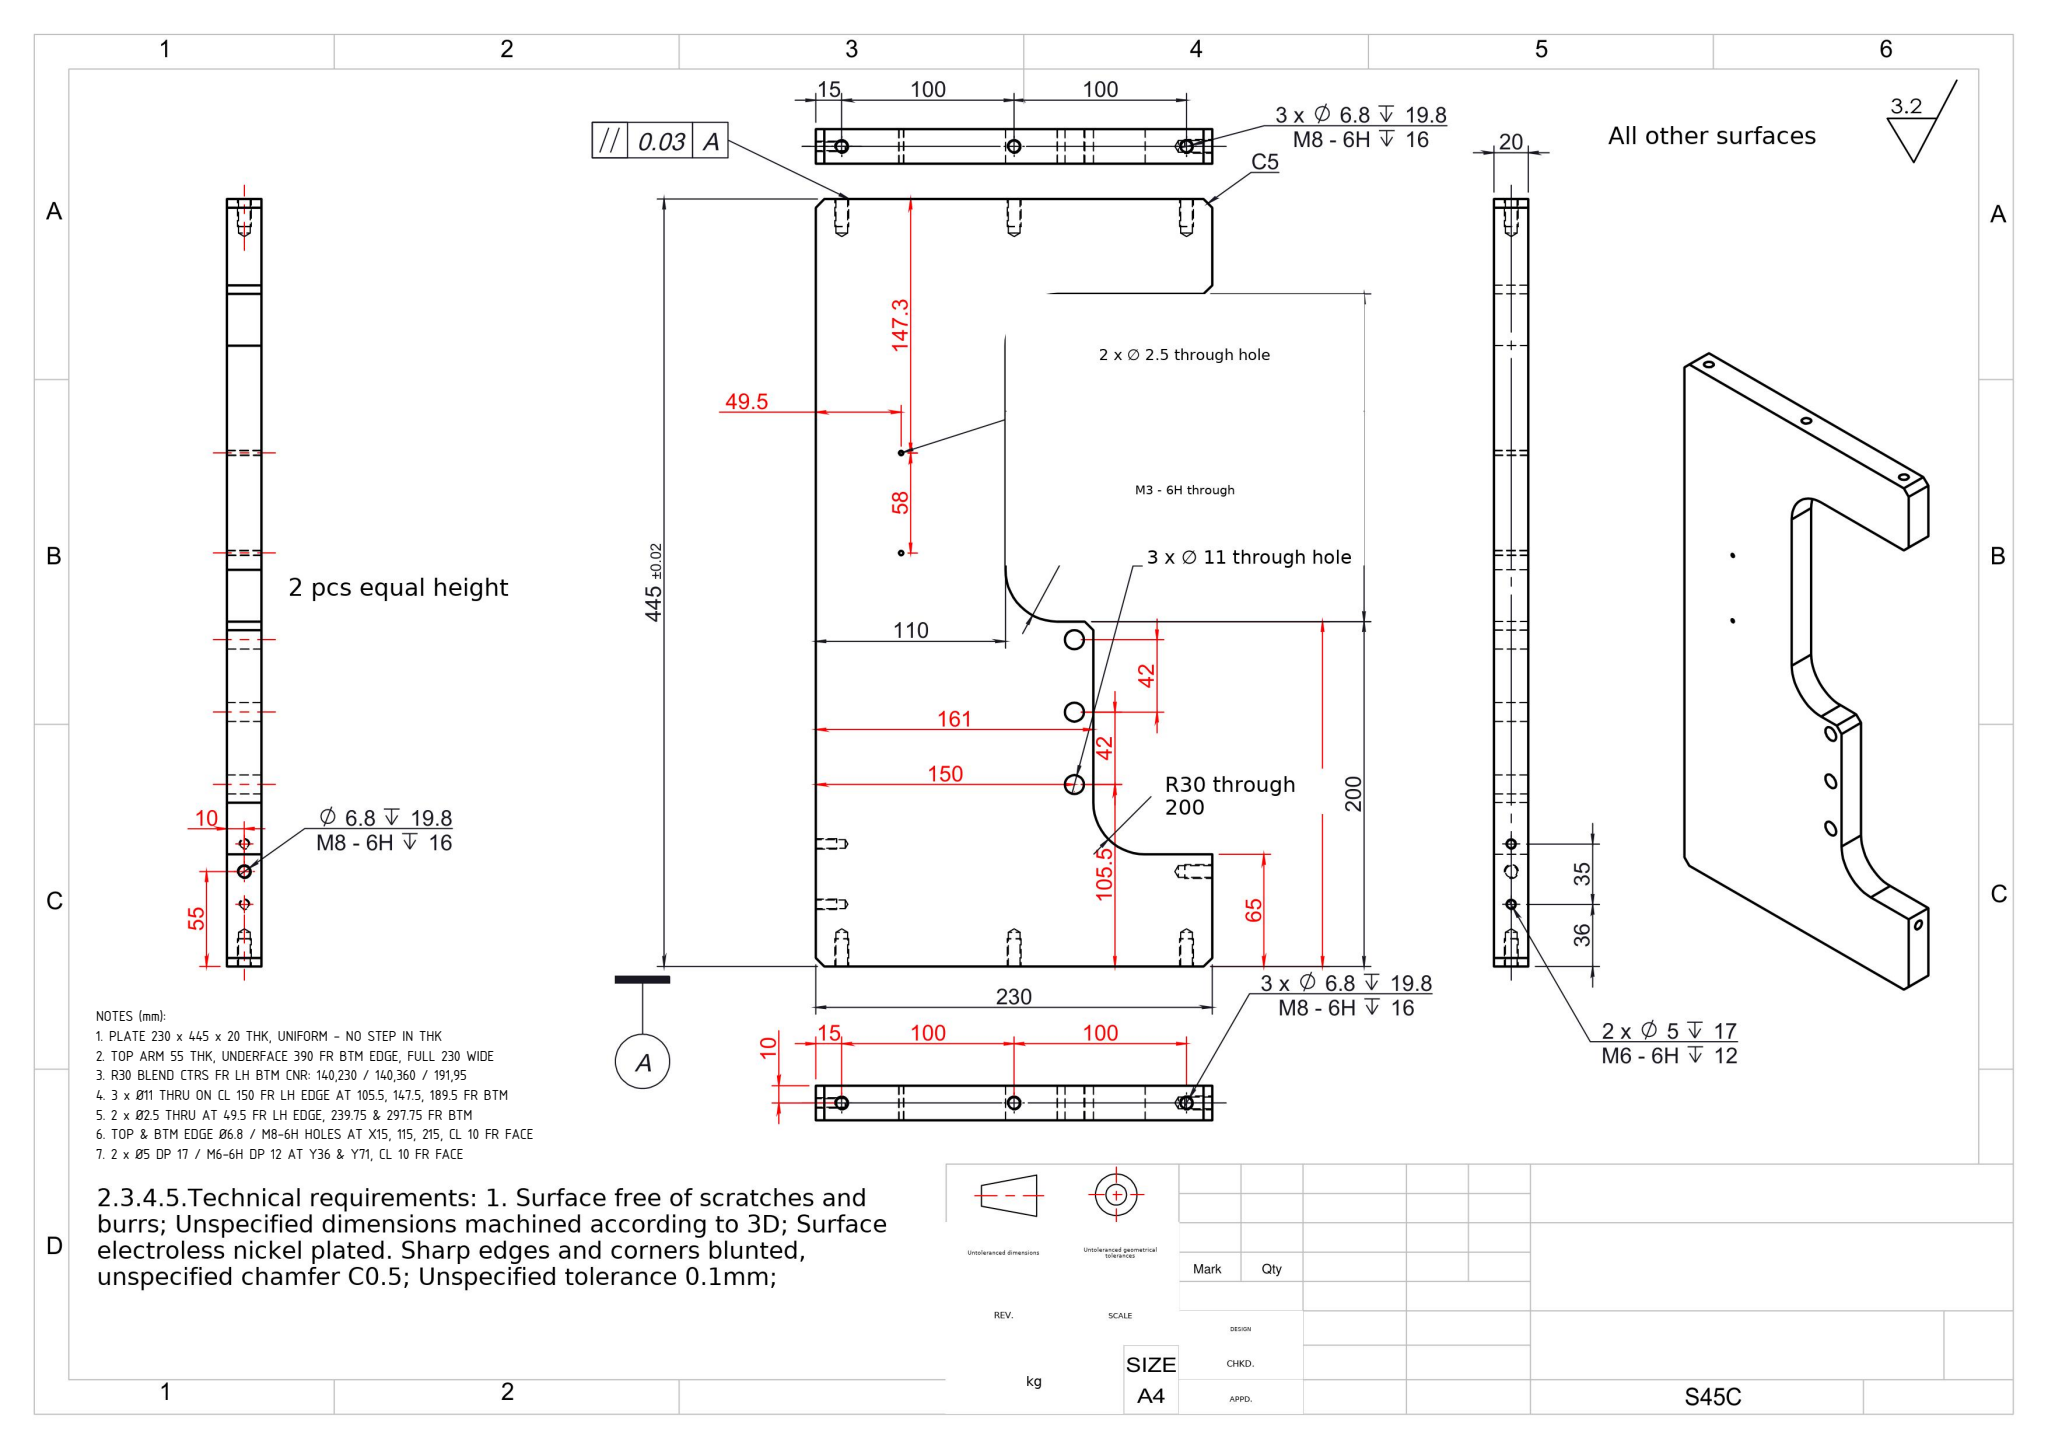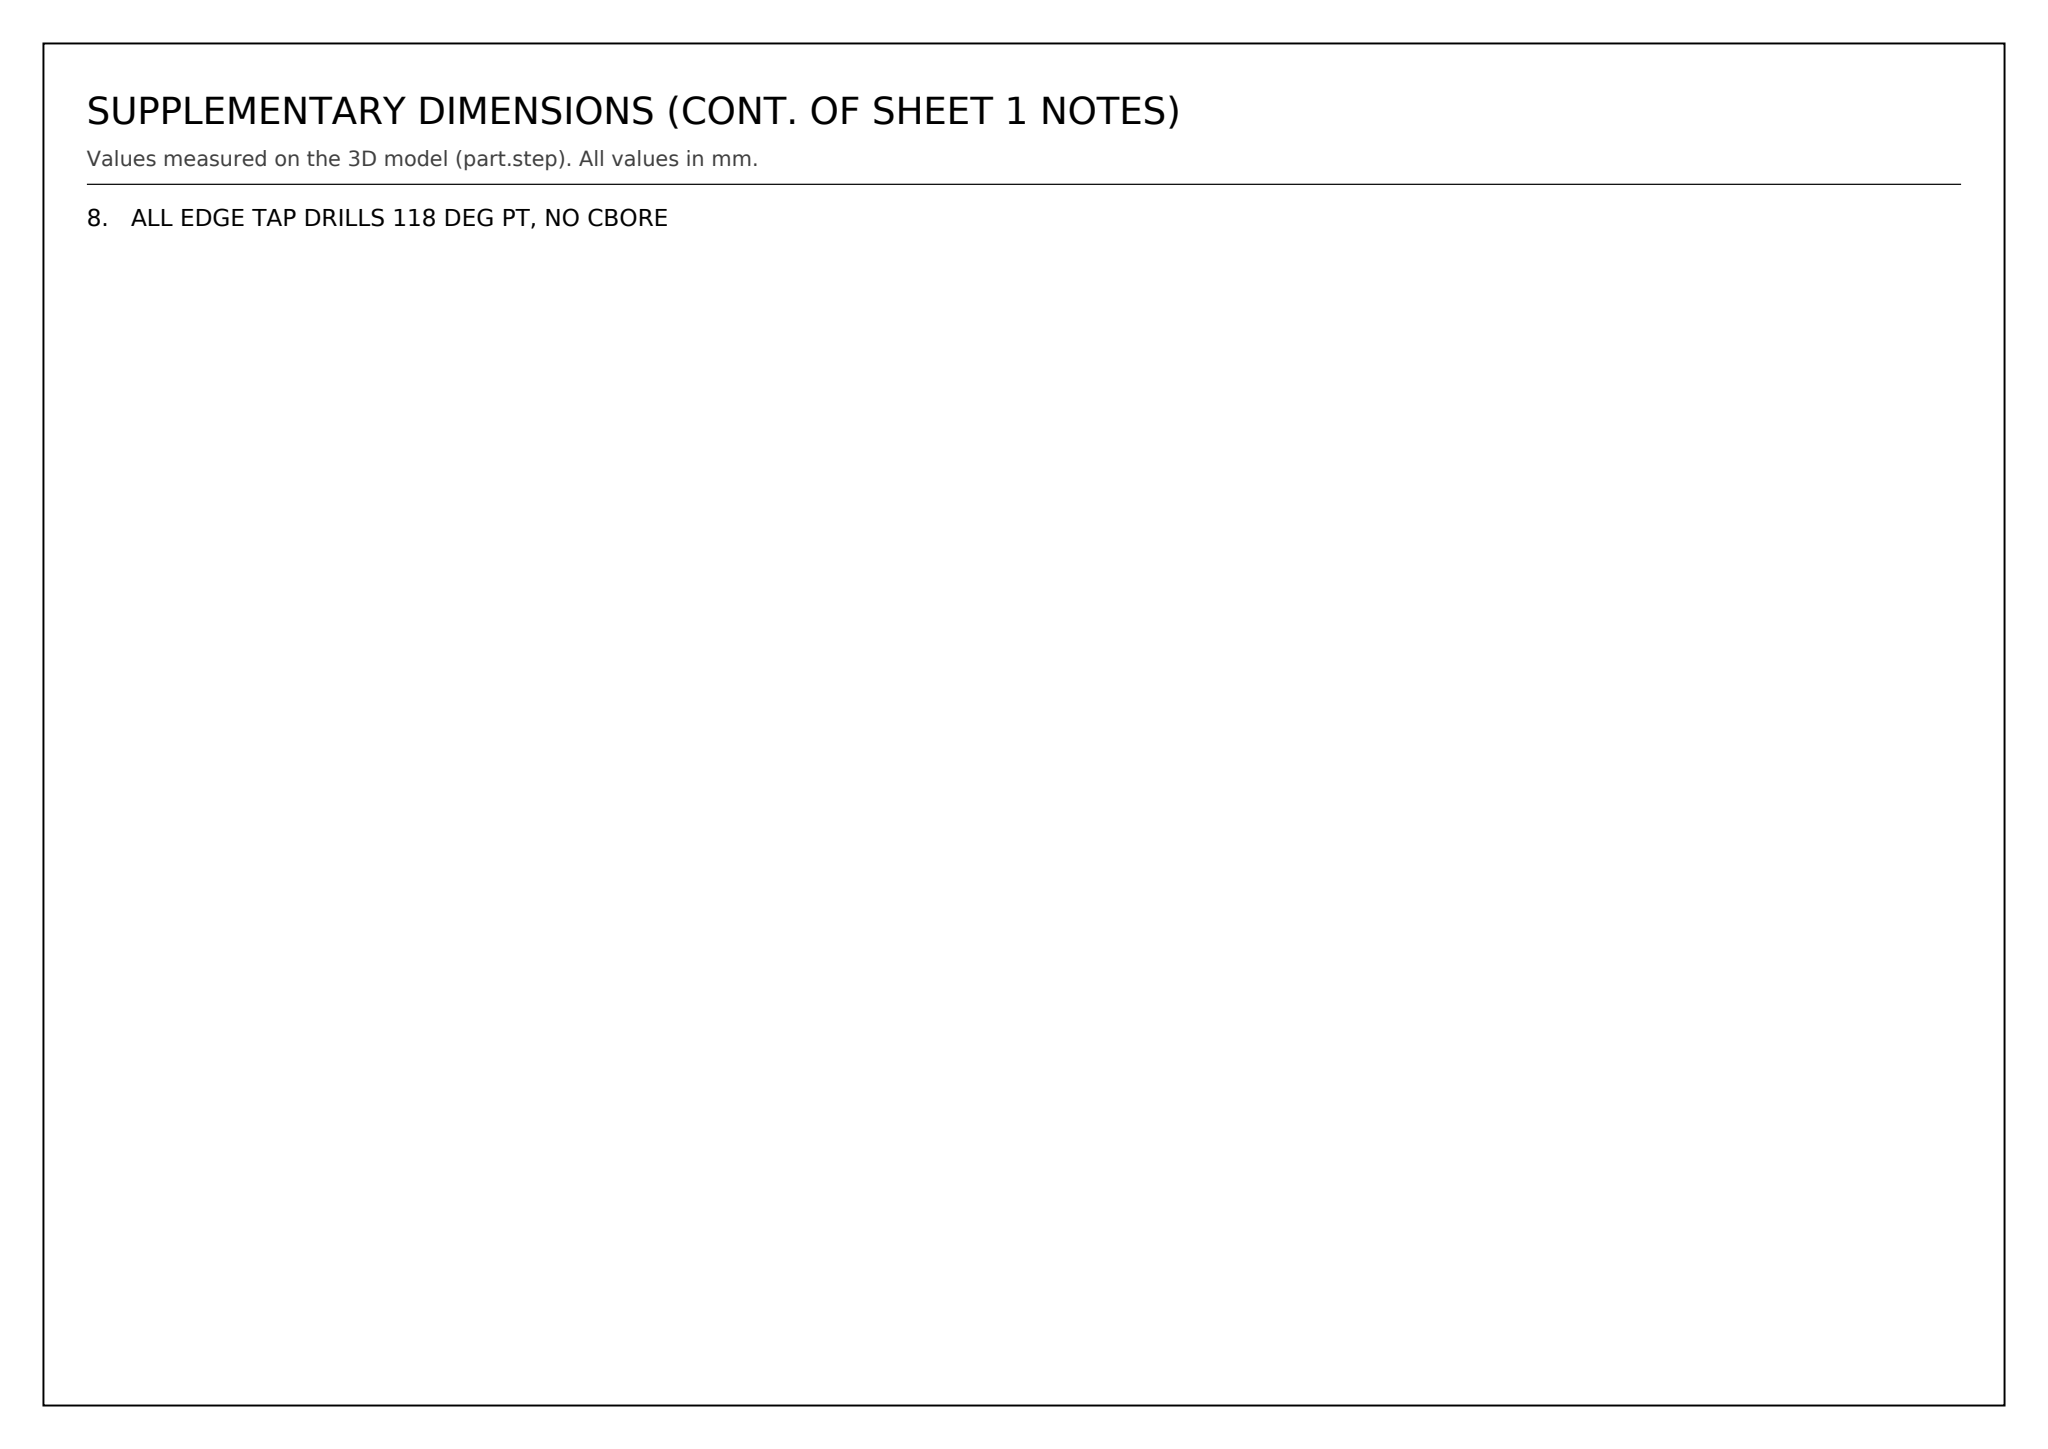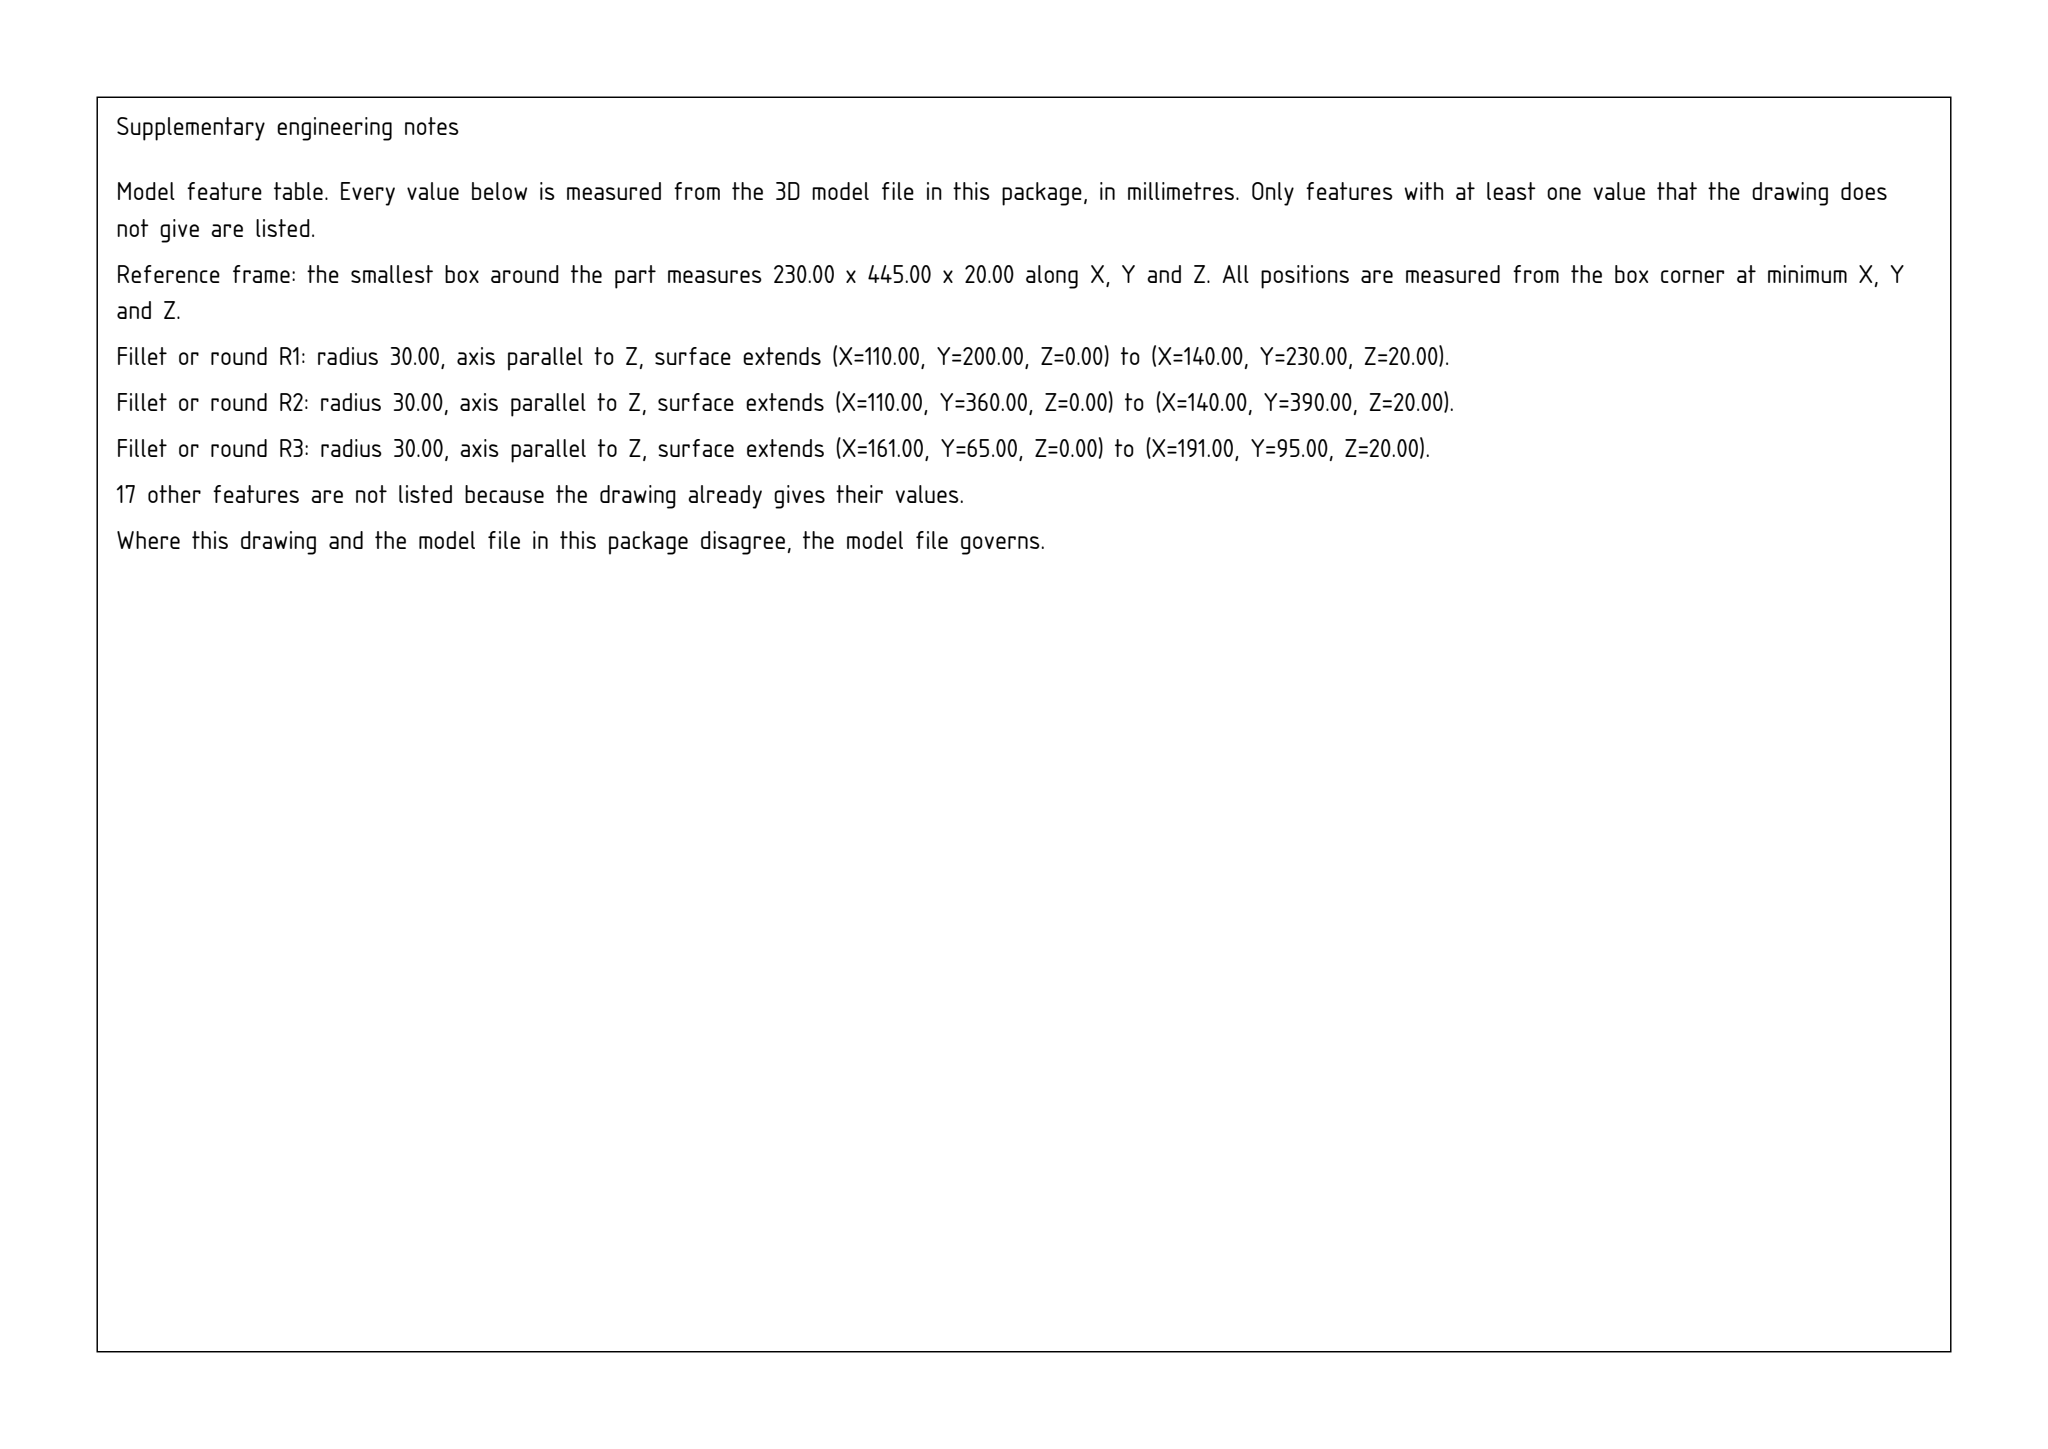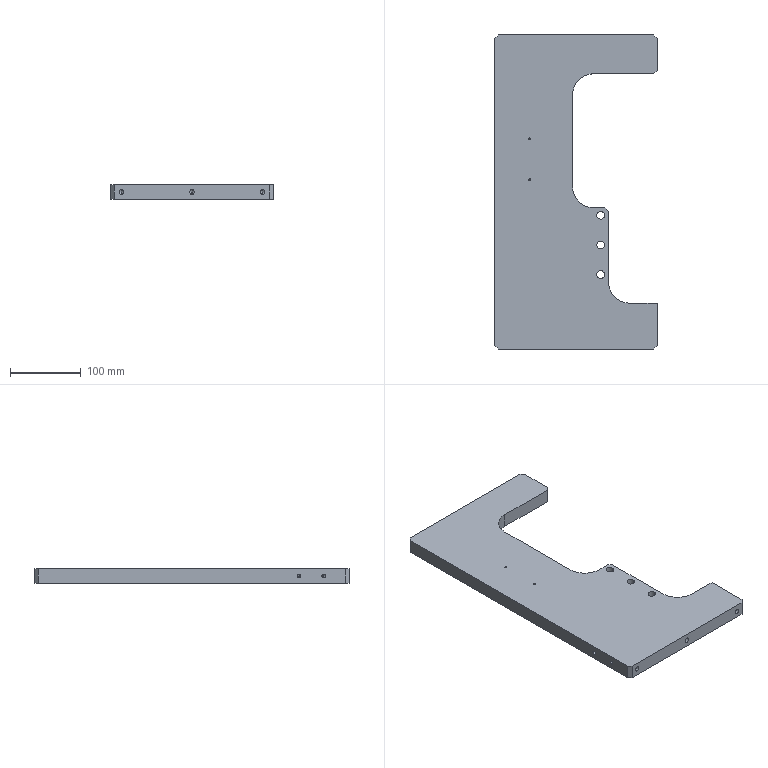Part | SolidWorks | mm | 1 solid | 67 faces | box 230 x 445 x 20 mm | volume 1403009 mm3 | cylinder 31 | cone 18 | plane 18 | commonest cylinder face diameters 6.8 x14 11 x6 2.5 x4 5 x4 60 x3
Drawing notes:
PLATE 230 x 445 x 20 THK, UNIFORM - NO STEP IN THK | from the solid: bbox 230x445x20; z-planes only at 0 and 20
TOP ARM 55 THK, UNDERFACE 390 FR BTM EDGE, FULL 230 WIDE | from the solid: y-planes 390 and 445; x-plane 230 (2 faces)
R30 BLEND CTRS FR LH BTM CNR: 140,230 / 140,360 / 191,95 | from the solid: Ø60 z-axis cyls at (140,230),(140,360),(191,95), L=20
3 x Ø11 THRU ON CL 150 FR LH EDGE AT 105.5, 147.5, 189.5 FR BTM | from the solid: Ø11 z-axis cyls at (150,105.5),(150,147.5),(150,189.5), L=20 full thk
2 x Ø2.5 THRU AT 49.5 FR LH EDGE, 239.75 & 297.75 FR BTM | from the solid: Ø2.5 z-axis cyls at (49.5,239.75),(49.5,297.75), L=20
TOP & BTM EDGE Ø6.8 / M8-6H HOLES AT X15, 115, 215, CL 10 FR FACE | from the solid: Ø6.8 y-axis cyls at x=15,115,215, z=10, L=19.75
2 x Ø5 DP 17 / M6-6H DP 12 AT Y36 & Y71, CL 10 FR FACE | from the solid: Ø5 x-axis cyls at y=36 and y=71, z=10, L=17
ALL EDGE TAP DRILLS 118 DEG PT, NO CBORE | from the solid: 118° cones ref Ø6.8 (14) and Ø5 (4); no larger bores
build123d program:
from build123d import *

# Parameters (mm, degrees)
SKETCH1_W             = 230
SKETCH1_H             = 445
BOSS_EXTRUDE1_DEPTH   = 10
SKETCH2_W             = 120
SKETCH2_H             = 190
CUT_EXTRUDE1_DEPTH    = 252.259
FILLET1_R             = 30
M8_TAPPED_HOLE1_D     = 6.8
M8_TAPPED_HOLE1_DEPTH = 19.75
M8_TAPPED_HOLE1_TIP   = 2.043
M8_TAPPED_HOLE2_D     = 6.8
M8_TAPPED_HOLE2_DEPTH = 19.75
M8_TAPPED_HOLE2_TIP   = 2.043
M6_TAPPED_HOLE1_D     = 5
M6_TAPPED_HOLE1_DEPTH = 17
M6_TAPPED_HOLE1_TIP   = 1.502
CHAMFER1_SIZE         = 5
SKETCH9_W             = 114.831
SKETCH9_H             = 135
CUT_EXTRUDE2_DEPTH    = 252.259
FILLET2_R             = 30
M8_TAPPED_HOLE3_D     = 6.8
M8_TAPPED_HOLE3_DEPTH = 19.75
M8_TAPPED_HOLE3_TIP   = 2.043
M10_CLEARANCE_HOLE1_D = 11
CHAMFER2_SIZE         = 5
M3_TAPPED_HOLE1_D     = 2.5


with BuildPart() as part:
    # Sketch1 → Boss-Extrude1 (new, symmetric)
    with BuildSketch(Plane.XY):
        Rectangle(SKETCH1_W, SKETCH1_H)
    extrude(amount=BOSS_EXTRUDE1_DEPTH, both=True)

    # Sketch2 → Cut-Extrude1 (cut, through all)
    with BuildSketch(Plane.XY.offset(10)):
        with Locations((55, 72.5)):
            Rectangle(SKETCH2_W, SKETCH2_H)
    extrude(amount=-CUT_EXTRUDE1_DEPTH, mode=Mode.SUBTRACT)

    # Fillet1
    fillet1_edges = [part.edges().sort_by_distance(p)[0] for p in [
        (-5, -22.5, 0),
        (-5, 167.5, 0),
    ]]
    fillet(fillet1_edges, radius=FILLET1_R)

    # M8 Tapped Hole1
    with Locations(Plane(origin=(0, 222.5, 0), x_dir=(1, 0, 0), z_dir=(0, 1, 0))):
        with Locations((100, 0), (-100, 0), (0, 0)):
            Hole(M8_TAPPED_HOLE1_D / 2, depth=M8_TAPPED_HOLE1_DEPTH)
            with Locations((0, 0, -(M8_TAPPED_HOLE1_DEPTH + M8_TAPPED_HOLE1_TIP / 2))):  # 118° drill point
                Cone(0, M8_TAPPED_HOLE1_D / 2, M8_TAPPED_HOLE1_TIP, mode=Mode.SUBTRACT)

    # M8 Tapped Hole2
    with Locations(Plane(origin=(0, -222.5, 0), x_dir=(-1, 0, 0), z_dir=(0, -1, 0))):
        with Locations((100, 0), (-100, 0), (0, 0)):
            Hole(M8_TAPPED_HOLE2_D / 2, depth=M8_TAPPED_HOLE2_DEPTH)
            with Locations((0, 0, -(M8_TAPPED_HOLE2_DEPTH + M8_TAPPED_HOLE2_TIP / 2))):  # 118° drill point
                Cone(0, M8_TAPPED_HOLE2_D / 2, M8_TAPPED_HOLE2_TIP, mode=Mode.SUBTRACT)

    # M6 Tapped Hole1
    with Locations(Plane.ZY.offset(115)):
        with Locations((0, -151.5), (0, -186.5)):
            Hole(M6_TAPPED_HOLE1_D / 2, depth=M6_TAPPED_HOLE1_DEPTH)
            with Locations((0, 0, -(M6_TAPPED_HOLE1_DEPTH + M6_TAPPED_HOLE1_TIP / 2))):  # 118° drill point
                Cone(0, M6_TAPPED_HOLE1_D / 2, M6_TAPPED_HOLE1_TIP, mode=Mode.SUBTRACT)

    # Chamfer1
    chamfer1_edges = [part.edges().sort_by_distance(p)[0] for p in [
        (115, 167.5, 0),
        (115, -22.5, 0),
        (-115, 222.5, 0),
        (115, 222.5, 0),
        (115, -222.5, 0),
        (-115, -222.5, 0),
    ]]
    chamfer(chamfer1_edges, length=CHAMFER1_SIZE)

    # Sketch9 → Cut-Extrude2 (cut, through all)
    with BuildSketch(Plane(origin=(0, 0, -10), x_dir=(-1, 0, 0), z_dir=(0, 0, -1))):
        with Locations((-103.415, -90)):
            Rectangle(SKETCH9_W, SKETCH9_H)
    extrude(amount=-CUT_EXTRUDE2_DEPTH, mode=Mode.SUBTRACT)

    # Fillet2
    fillet2_edges = [part.edges().sort_by_distance(p)[0] for p in [
        (46, -157.5, 0),
    ]]
    fillet(fillet2_edges, radius=FILLET2_R)

    # M8 Tapped Hole3
    with Locations(Plane(origin=(115, 0, 0), x_dir=(0, 0, -1), z_dir=(1, 0, 0))):
        with Locations((0, -167.5)):
            Hole(M8_TAPPED_HOLE3_D / 2, depth=M8_TAPPED_HOLE3_DEPTH)
            with Locations((0, 0, -(M8_TAPPED_HOLE3_DEPTH + M8_TAPPED_HOLE3_TIP / 2))):  # 118° drill point
                Cone(0, M8_TAPPED_HOLE3_D / 2, M8_TAPPED_HOLE3_TIP, mode=Mode.SUBTRACT)

    # M10 Clearance Hole1 (through all)
    with Locations(Plane(origin=(0, 0, -10), x_dir=(-1, 0, 0), z_dir=(0, 0, -1))):
        with Locations((-35, -117), (-35, -75), (-35, -33)):
            Hole(M10_CLEARANCE_HOLE1_D / 2)

    # Chamfer2
    chamfer2_edges = [part.edges().sort_by_distance(p)[0] for p in [
        (46, -22.5, 0),
    ]]
    chamfer(chamfer2_edges, length=CHAMFER2_SIZE)

    # M3 Tapped Hole1 (through all)
    with Locations(Plane(origin=(0, 0, -10), x_dir=(-1, 0, 0), z_dir=(0, 0, -1))):
        with Locations((65.5, 17.25), (65.5, 75.25)):
            Hole(M3_TAPPED_HOLE1_D / 2)


solid = part.part